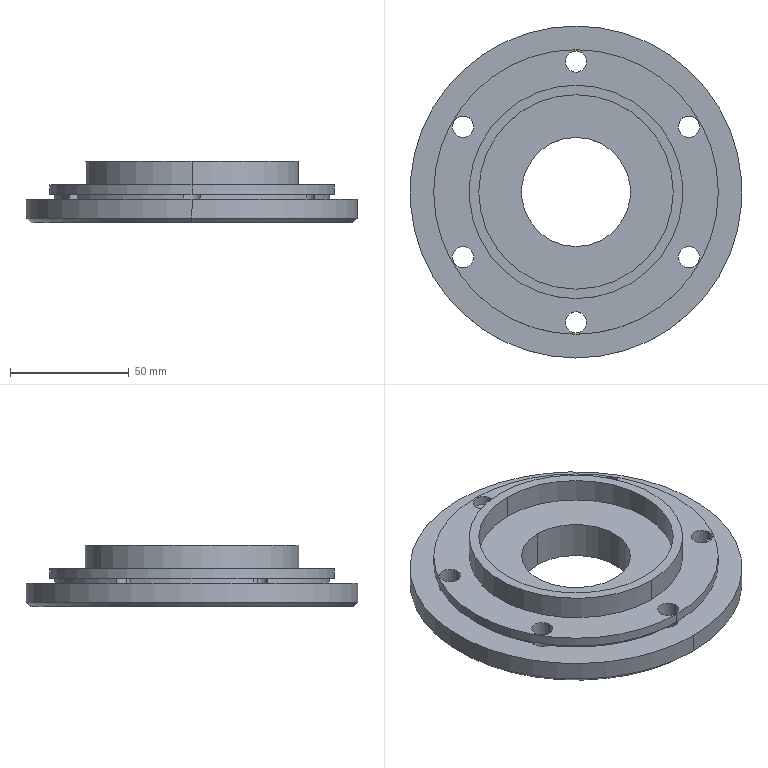Component | SolidWorks | OutputAxisEndCover2-0718-1 | 1 solid | 36 faces | box 140 x 140 x 26 mm | volume 197638 mm3 | cylinder 28 | plane 6 | cone 2 | commonest cylinder face diameters 9 x12 116 x6 46 x2 82 x2 90 x2 140 x2 120 x2
build123d program:
from build123d import *

# Parameters (mm, degrees)
SKETCH2_R                  = 45
BOSS_EXTRUDE1_DEPTH        = 10
SKETCH6_R                  = 41
CUT_EXTRUDE1_DEPTH         = 10
F_8_5_8_5_DIAMETER_HOLE1_D = 9
CIRPATTERN1_COUNT          = 6
CHAMFER1_SIZE              = 2
SKETCH7_R                  = 23
CUT_EXTRUDE2_DEPTH         = 20


with BuildPart() as part:
    # Sketch1 → Revolve1 (revolve)
    with BuildSketch(Plane(origin=(0, 0, 0), x_dir=(-1, 0, 0), z_dir=(0, 0, -1)), mode=Mode.PRIVATE) as revolve1_sk:
        Polygon((-6, 60), (-6, 0), (10, 0), (10, 70), (0, 70), (0, 58), (-2, 58), (-2, 60), align=None)
    revolve(revolve1_sk.sketch.rotate(Axis((6, 0, 0), (-1, 0, 0)), 180), axis=Axis((6, 0, 0), (-1, 0, 0)))

    # Sketch2 → Boss-Extrude1 (add)
    with BuildSketch(Plane(origin=(6, 0, 0), x_dir=(0, 0, -1), z_dir=(1, 0, 0))):
        with Locations(Location((0, 0, 0), (0, 0, 90))):
            Circle(SKETCH2_R)
    extrude(amount=BOSS_EXTRUDE1_DEPTH)

    # Sketch6 → Cut-Extrude1 (cut)
    with BuildSketch(Plane(origin=(16, 0, 0), x_dir=(0, 0, -1), z_dir=(1, 0, 0))):
        with Locations(Location((0, 0, 0), (0, 0, 90))):
            Circle(SKETCH6_R)
    extrude(amount=-CUT_EXTRUDE1_DEPTH, mode=Mode.SUBTRACT)

    # 8.5 _8.5_ Diameter Hole1 (through all)
    with Locations(Plane.ZY.offset(10)):
        with Locations((0, 55)):
            f_8_5_8_5_diameter_hole1 = Hole(F_8_5_8_5_DIAMETER_HOLE1_D / 2)

    # CirPattern1: 8.5 _8.5_ Diameter Hole1 ×6 about axis
    cirpattern1_axis = Axis((0, 0, 0), (1, 0, 0))
    for i in range(1, CIRPATTERN1_COUNT):
        add(f_8_5_8_5_diameter_hole1.rotate(cirpattern1_axis, i * 360 / CIRPATTERN1_COUNT), mode=Mode.SUBTRACT)

    # Chamfer1
    chamfer1_edges = [part.edges().sort_by_distance(p)[0] for p in [
        (-10, 70, 0),
    ]]
    chamfer(chamfer1_edges, length=CHAMFER1_SIZE)

    # Sketch7 → Cut-Extrude2 (cut)
    with BuildSketch(Plane.ZY.offset(10)):
        with Locations(Location((0, 0, 0), (0, 0, 270))):
            Circle(SKETCH7_R)
    extrude(amount=-CUT_EXTRUDE2_DEPTH, mode=Mode.SUBTRACT)


solid = part.part

# Placed as in the assembly
solid = solid.moved(Location((-30, 0, -153), (0, -90, 0)))